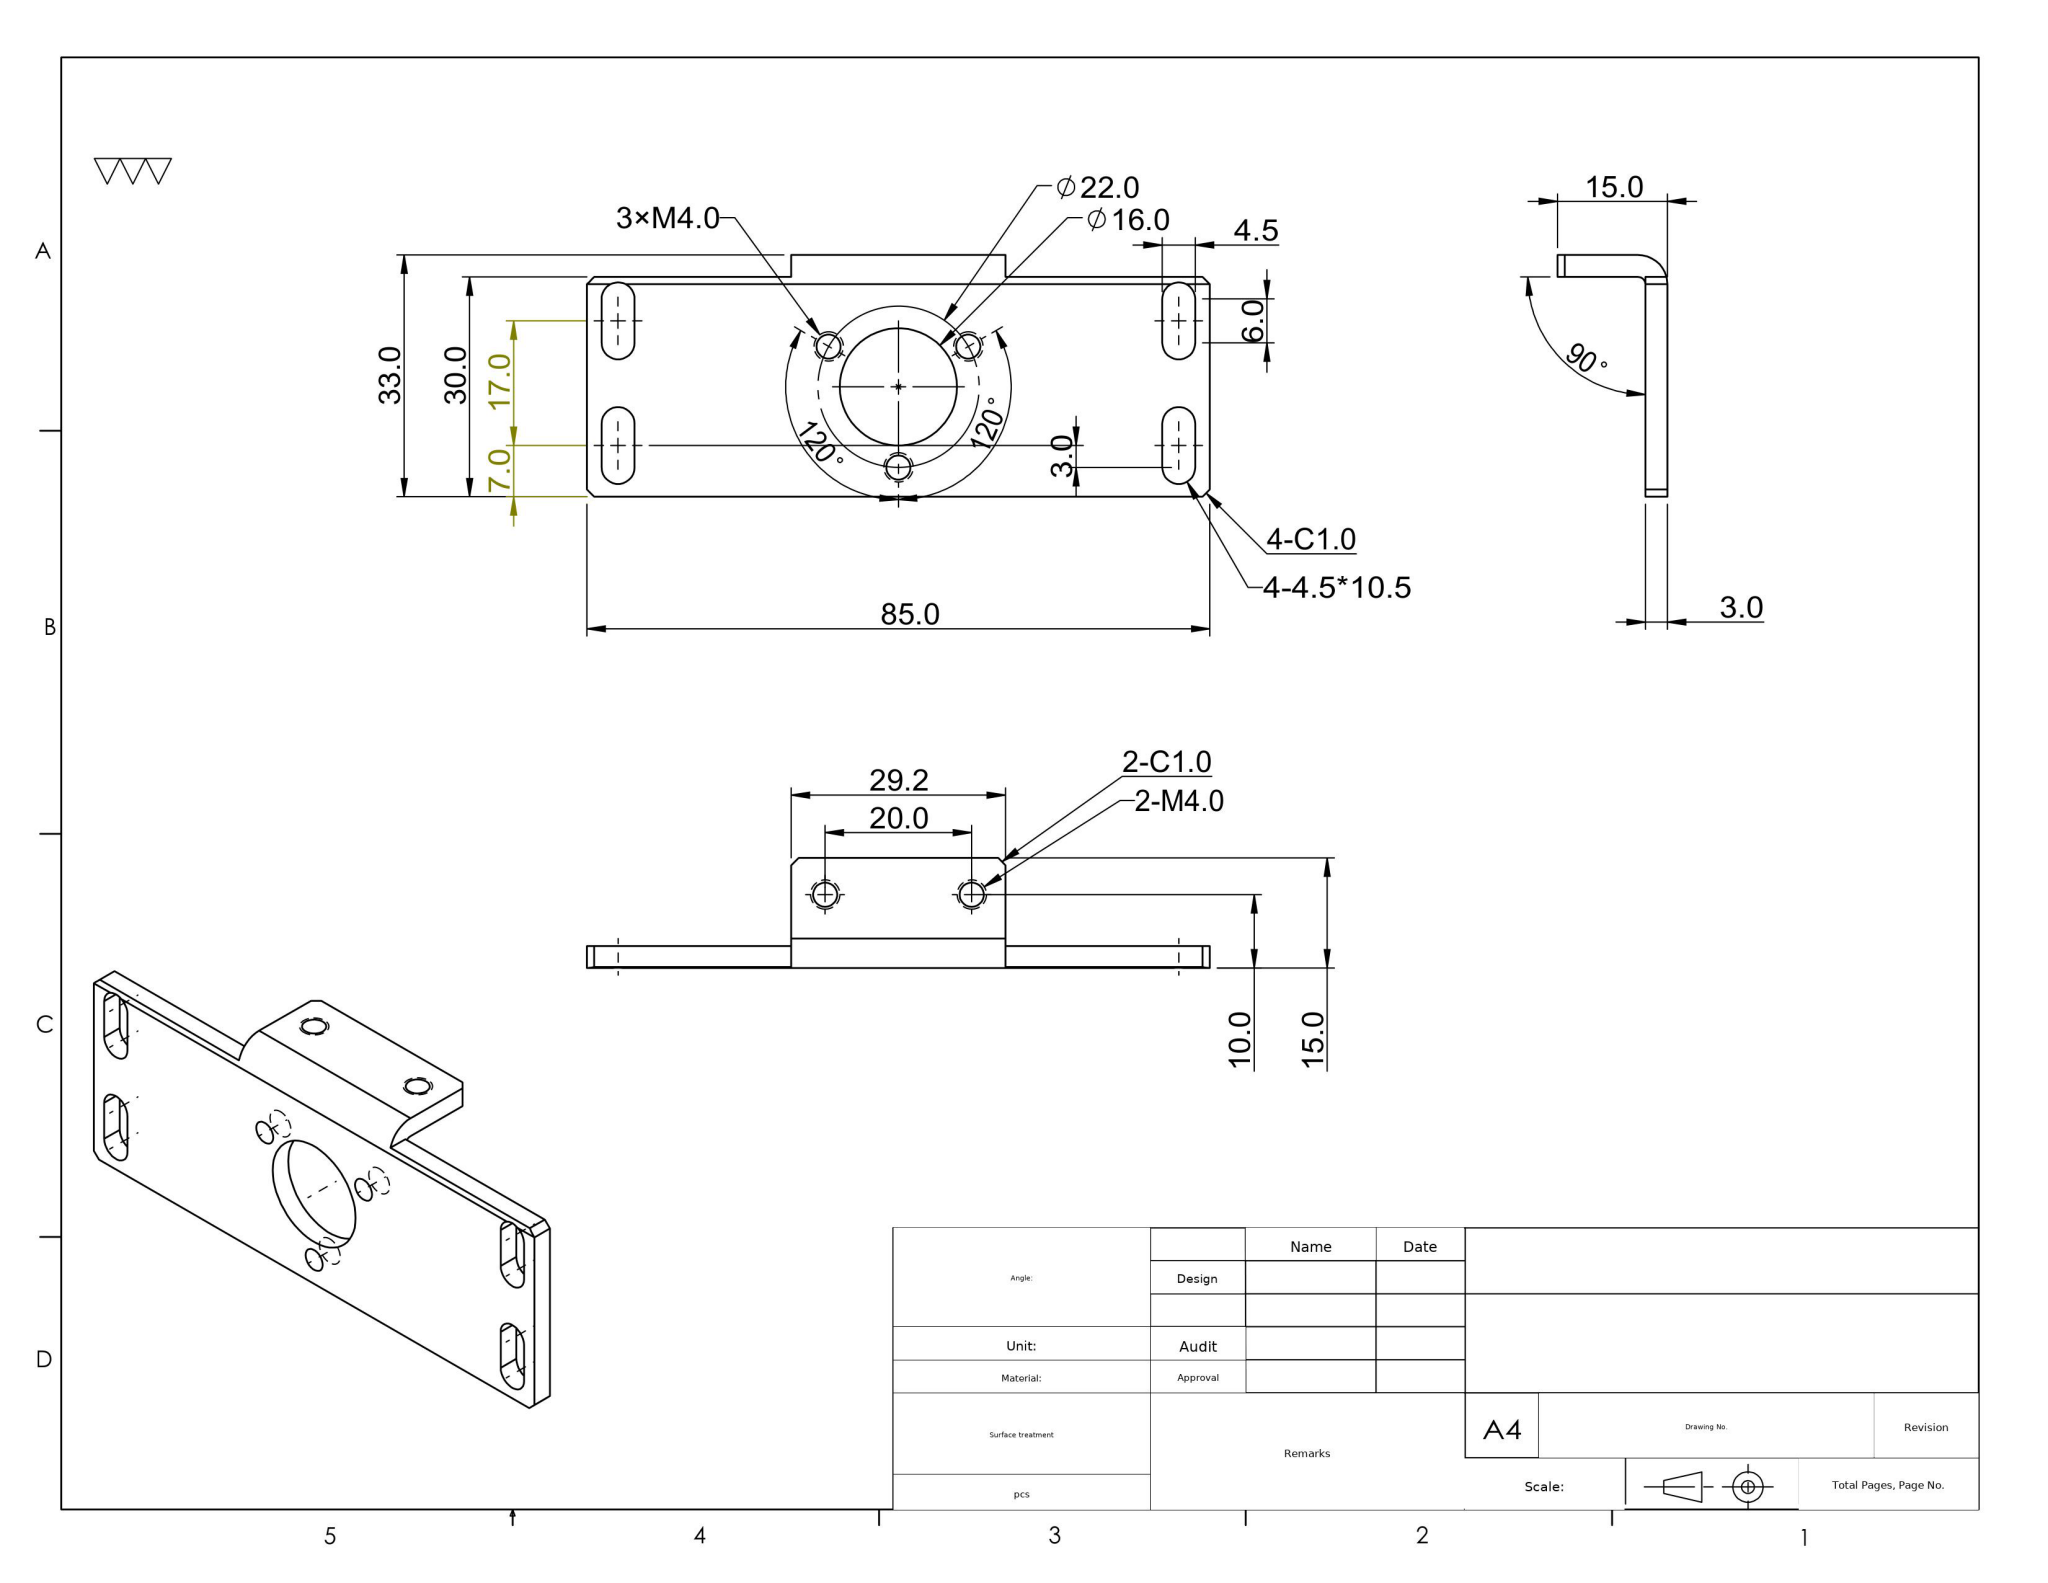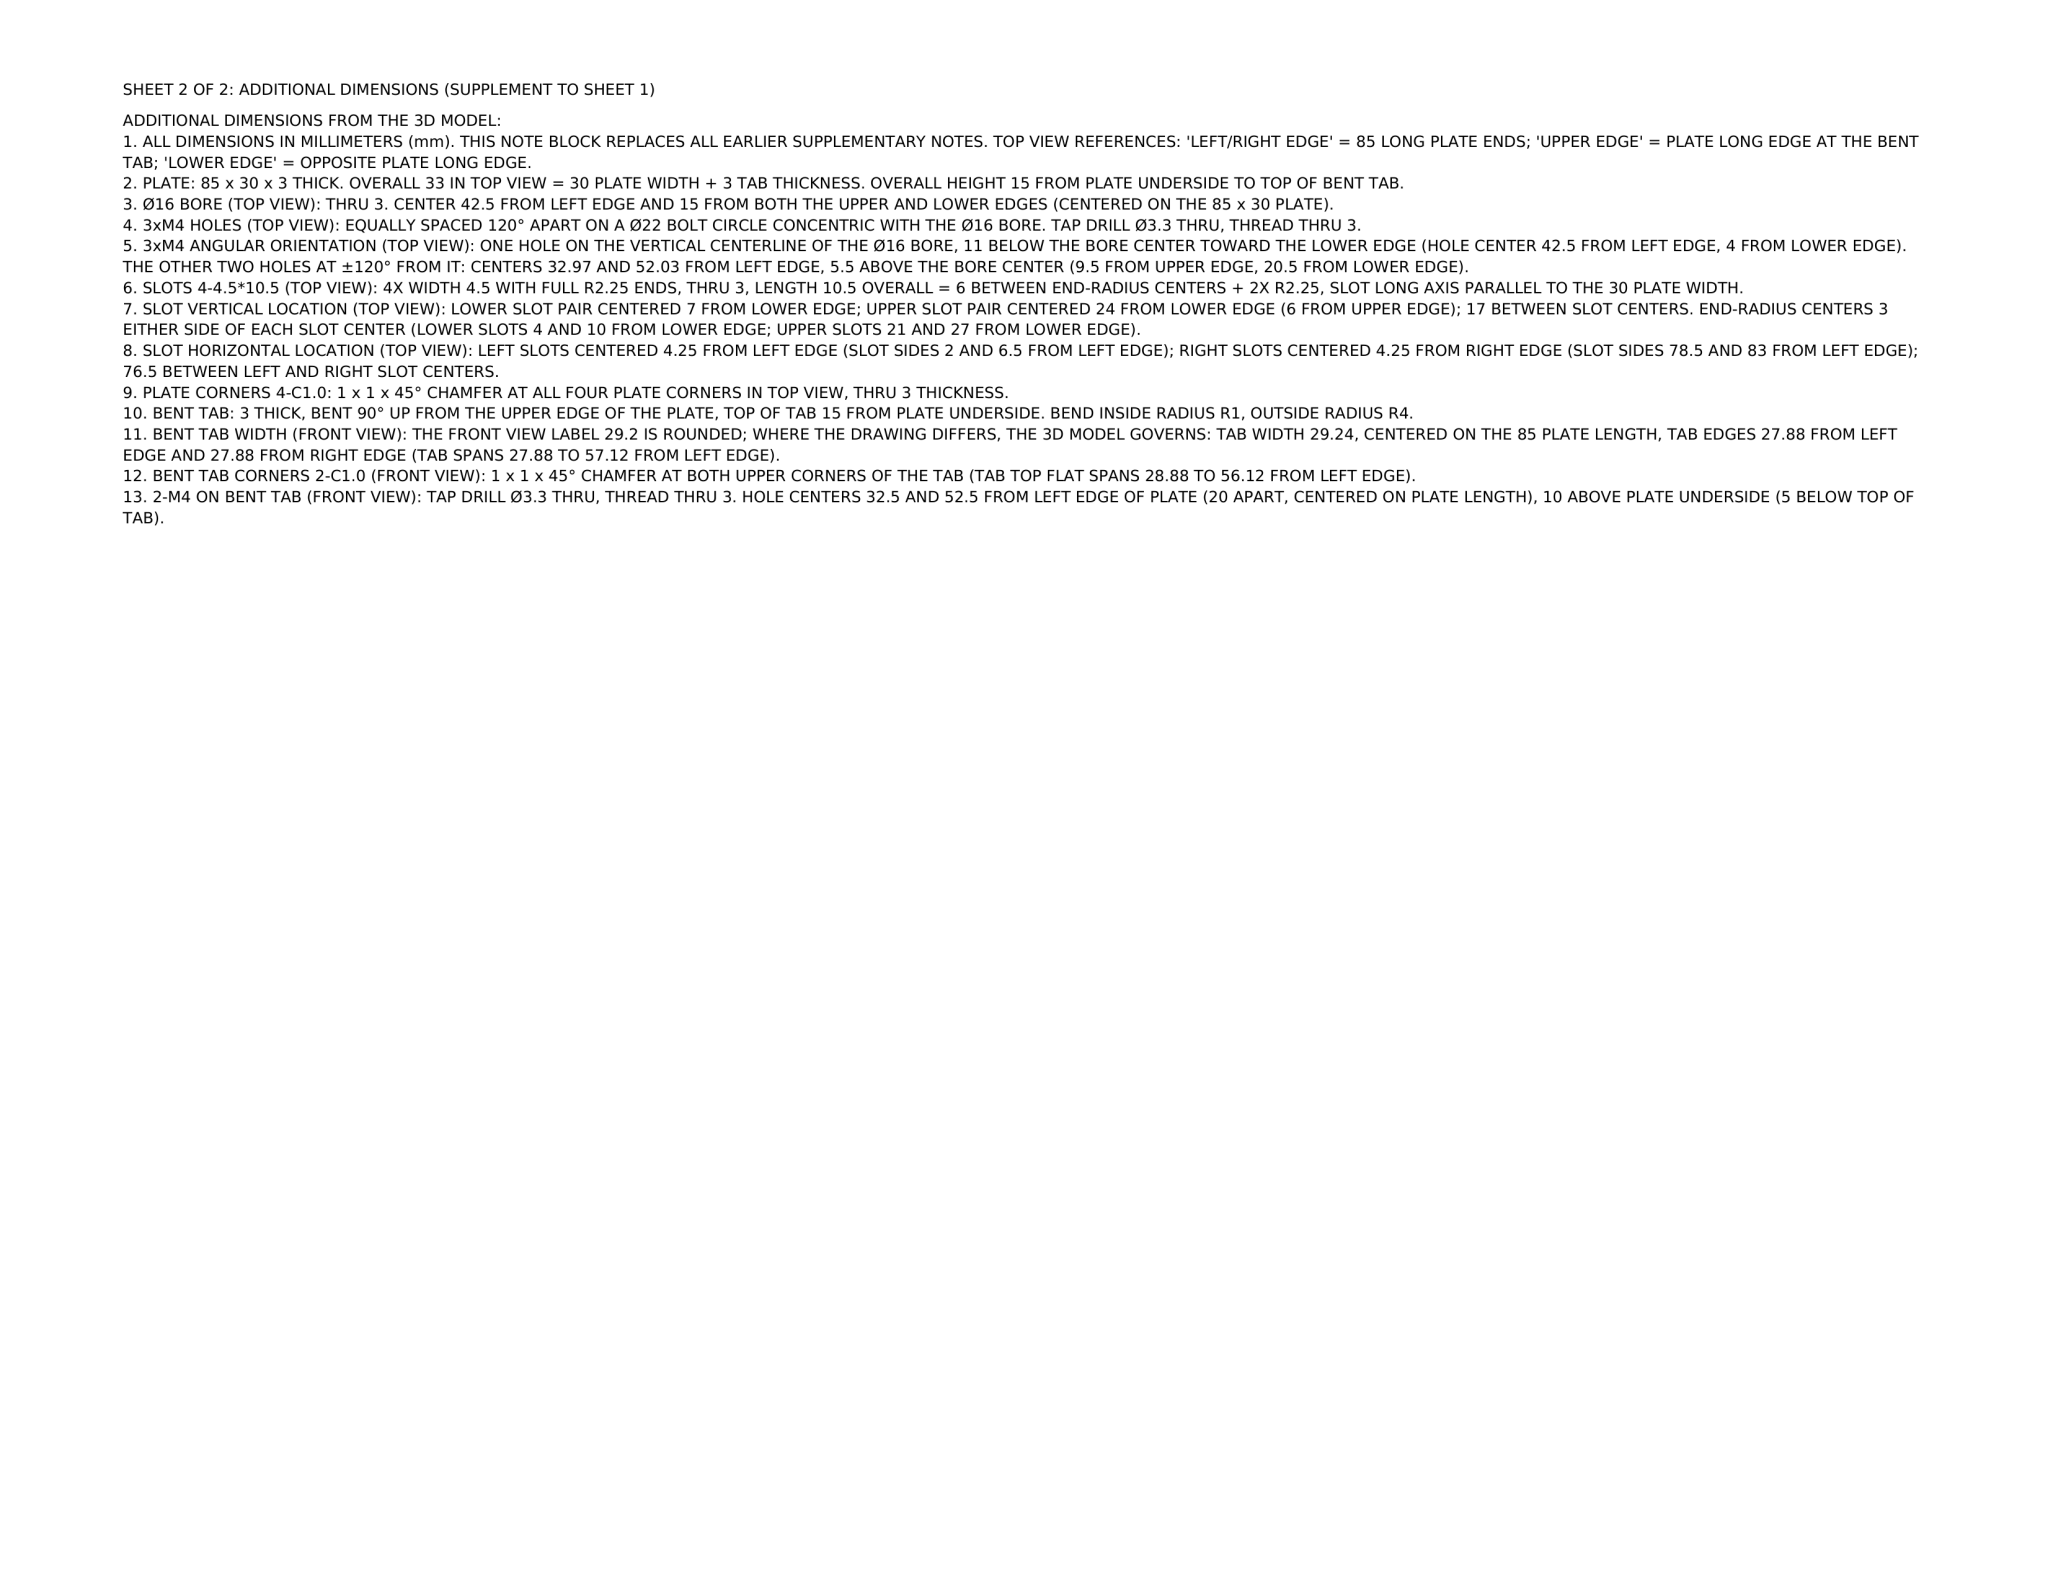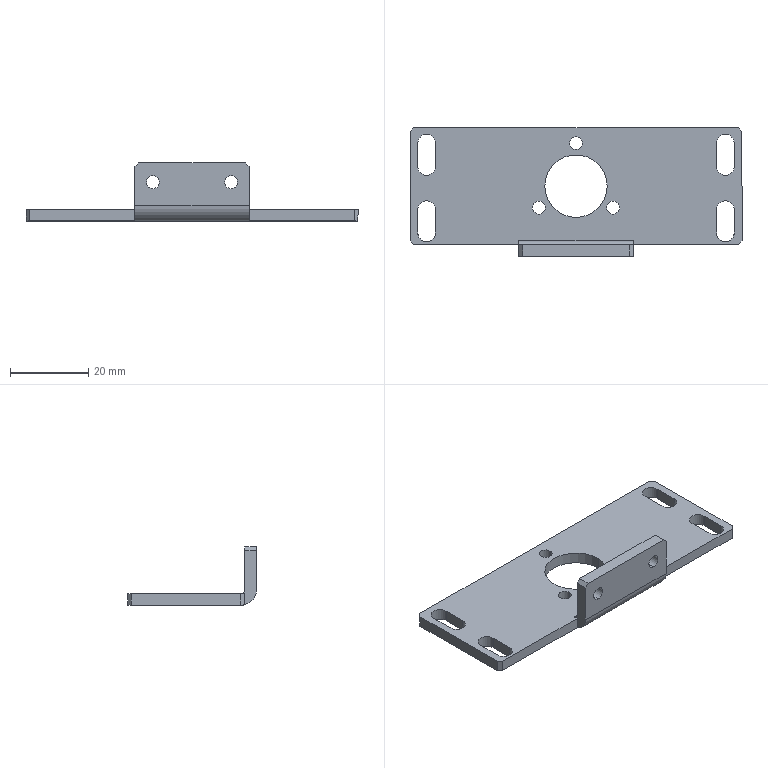Part | NX | mm | 1 solid | 48 faces | box 85 x 33 x 15 mm | volume 7614 mm3 | plane 26 | cylinder 22 | commonest cylinder face diameters 3.3 x10 4.5 x8 16 x2 8 x1 2 x1